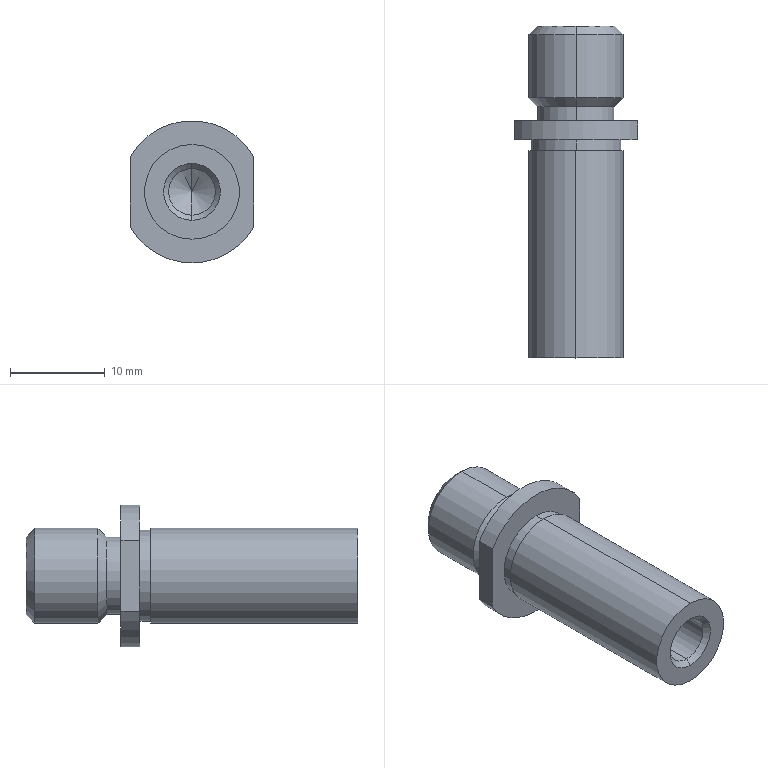Component | SolidWorks | MDJ12-10-Y2-F23-E10-N6.stp-1 | 1 solid | 28 faces | box 13 x 35 x 15 mm | volume 2570 mm3 | cylinder 13 | cone 8 | plane 7 | commonest cylinder face diameters 10 x4 15 x3 4.917 x2 8.16 x2 9.6 x2 | material 45
STEP:
#1=COLOUR_RGB('',0.7922,0.8196,0.9333);
#2=FILL_AREA_STYLE_COLOUR('',#1);
#3=FILL_AREA_STYLE('',(#2));
#4=SURFACE_STYLE_FILL_AREA(#3);
#5=SURFACE_SIDE_STYLE('',(#4));
#6=SURFACE_STYLE_USAGE(.BOTH.,#5);
#7=PRESENTATION_STYLE_ASSIGNMENT((#6));
#8=CARTESIAN_POINT('',(0.2836,0.06236,15.932));
#9=VERTEX_POINT('',#8);
#10=CARTESIAN_POINT('',(0.2836,0.06236,16.253));
#11=VERTEX_POINT('',#10);
#12=CARTESIAN_POINT('',(0.2836,0.06236,16.092));
#13=DIRECTION('',(-0.,-1.,0.));
#14=DIRECTION('',(-0.,0.,-1.));
#15=AXIS2_PLACEMENT_3D('',#12,#13,#14);
#16=CIRCLE('',#15,0.1606);
#17=EDGE_CURVE('',#9,#11,#16,.T.);
#18=ORIENTED_EDGE('',*,*,#17,.F.);
#19=CARTESIAN_POINT('',(0.2836,0.09858,15.896));
#20=VERTEX_POINT('',#19);
#21=CARTESIAN_POINT('',(0.2836,0.09858,15.896));
#22=DIRECTION('',(0.,0.7071,-0.7071));
#23=VECTOR('',#22,39.37);
#24=LINE('',#21,#23);
#25=EDGE_CURVE('',#9,#20,#24,.T.);
#26=ORIENTED_EDGE('',*,*,#25,.T.);
#27=CARTESIAN_POINT('',(0.2836,0.09858,16.289));
#28=VERTEX_POINT('',#27);
#29=CARTESIAN_POINT('',(0.2836,0.09858,16.092));
#30=DIRECTION('',(-0.,-1.,0.));
#31=DIRECTION('',(-0.,0.,-1.));
#32=AXIS2_PLACEMENT_3D('',#29,#30,#31);
#33=CIRCLE('',#32,0.1969);
#34=EDGE_CURVE('',#20,#28,#33,.T.);
#35=ORIENTED_EDGE('',*,*,#34,.T.);
#36=CARTESIAN_POINT('',(0.2836,0.09858,16.289));
#37=DIRECTION('',(0.,0.7071,0.7071));
#38=VECTOR('',#37,39.37);
#39=LINE('',#36,#38);
#40=EDGE_CURVE('',#11,#28,#39,.T.);
#41=ORIENTED_EDGE('',*,*,#40,.F.);
#42=EDGE_LOOP('',(#18,#26,#35,#41));
#43=FACE_OUTER_BOUND('',#42,.T.);
#44=CARTESIAN_POINT('',(0.2836,0.09858,16.092));
#45=DIRECTION('',(0.,1.,-0.));
#46=DIRECTION('',(0.,0.,1.));
#47=AXIS2_PLACEMENT_3D('',#44,#45,#46);
#48=CONICAL_SURFACE('',#47,0.1969,0.7854);
#49=ADVANCED_FACE('',(#43),#48,.T.);
#50=CARTESIAN_POINT('',(0.2836,-0.981,16.289));
#51=VERTEX_POINT('',#50);
#52=CARTESIAN_POINT('',(0.2836,-0.981,15.896));
#53=VERTEX_POINT('',#52);
#54=CARTESIAN_POINT('',(0.2836,-0.981,16.092));
#55=DIRECTION('',(-0.,-1.,0.));
#56=DIRECTION('',(-0.,0.,-1.));
#57=AXIS2_PLACEMENT_3D('',#54,#55,#56);
#58=CIRCLE('',#57,0.1969);
#59=EDGE_CURVE('',#51,#53,#58,.T.);
#60=ORIENTED_EDGE('',*,*,#59,.F.);
#61=CARTESIAN_POINT('',(0.2836,-0.1207,16.289));
#62=VERTEX_POINT('',#61);
#63=CARTESIAN_POINT('',(0.2836,-0.981,16.289));
#64=DIRECTION('',(0.,1.,-0.));
#65=VECTOR('',#64,39.37);
#66=LINE('',#63,#65);
#67=EDGE_CURVE('',#51,#62,#66,.T.);
#68=ORIENTED_EDGE('',*,*,#67,.T.);
#69=CARTESIAN_POINT('',(0.2836,-0.1207,15.896));
#70=VERTEX_POINT('',#69);
#71=CARTESIAN_POINT('',(0.2836,-0.1207,16.092));
#72=DIRECTION('',(-0.,-1.,0.));
#73=DIRECTION('',(-0.,0.,-1.));
#74=AXIS2_PLACEMENT_3D('',#71,#72,#73);
#75=CIRCLE('',#74,0.1969);
#76=EDGE_CURVE('',#62,#70,#75,.T.);
#77=ORIENTED_EDGE('',*,*,#76,.T.);
#78=CARTESIAN_POINT('',(0.2836,-0.981,15.896));
#79=DIRECTION('',(0.,1.,-0.));
#80=VECTOR('',#79,39.37);
#81=LINE('',#78,#80);
#82=EDGE_CURVE('',#53,#70,#81,.T.);
#83=ORIENTED_EDGE('',*,*,#82,.F.);
#84=EDGE_LOOP('',(#60,#68,#77,#83));
#85=FACE_OUTER_BOUND('',#84,.T.);
#86=CARTESIAN_POINT('',(0.2836,-0.981,16.092));
#87=DIRECTION('',(0.,1.,-0.));
#88=DIRECTION('',(-0.,0.,-1.));
#89=AXIS2_PLACEMENT_3D('',#86,#87,#88);
#90=CYLINDRICAL_SURFACE('',#89,0.1969);
#91=ADVANCED_FACE('',(#85),#90,.T.);
#92=CARTESIAN_POINT('',(0.2836,-0.9596,16.189));
#93=VERTEX_POINT('',#92);
#94=CARTESIAN_POINT('',(0.2836,-0.9596,15.996));
#95=VERTEX_POINT('',#94);
#96=CARTESIAN_POINT('',(0.2836,-0.9596,16.092));
#97=DIRECTION('',(-0.,-1.,0.));
#98=DIRECTION('',(-0.,0.,-1.));
#99=AXIS2_PLACEMENT_3D('',#96,#97,#98);
#100=CIRCLE('',#99,0.09679);
#101=EDGE_CURVE('',#93,#95,#100,.T.);
#102=ORIENTED_EDGE('',*,*,#101,.F.);
#103=CARTESIAN_POINT('',(0.2836,-0.981,16.211));
#104=VERTEX_POINT('',#103);
#105=CARTESIAN_POINT('',(0.2836,-0.981,16.211));
#106=DIRECTION('',(0.,-0.7071,0.7071));
#107=VECTOR('',#106,39.37);
#108=LINE('',#105,#107);
#109=EDGE_CURVE('',#93,#104,#108,.T.);
#110=ORIENTED_EDGE('',*,*,#109,.T.);
#111=CARTESIAN_POINT('',(0.2836,-0.981,15.974));
#112=VERTEX_POINT('',#111);
#113=CARTESIAN_POINT('',(0.2836,-0.981,16.092));
#114=DIRECTION('',(-0.,-1.,0.));
#115=DIRECTION('',(-0.,0.,-1.));
#116=AXIS2_PLACEMENT_3D('',#113,#114,#115);
#117=CIRCLE('',#116,0.1181);
#118=EDGE_CURVE('',#104,#112,#117,.T.);
#119=ORIENTED_EDGE('',*,*,#118,.T.);
#120=CARTESIAN_POINT('',(0.2836,-0.981,15.974));
#121=DIRECTION('',(-0.,-0.7071,-0.7071));
#122=VECTOR('',#121,39.37);
#123=LINE('',#120,#122);
#124=EDGE_CURVE('',#95,#112,#123,.T.);
#125=ORIENTED_EDGE('',*,*,#124,.F.);
#126=EDGE_LOOP('',(#102,#110,#119,#125));
#127=FACE_OUTER_BOUND('',#126,.T.);
#128=CARTESIAN_POINT('',(0.2836,-0.981,16.092));
#129=DIRECTION('',(-0.,-1.,0.));
#130=DIRECTION('',(-0.,0.,-1.));
#131=AXIS2_PLACEMENT_3D('',#128,#129,#130);
#132=CONICAL_SURFACE('',#131,0.1181,0.7854);
#133=ADVANCED_FACE('',(#127),#132,.F.);
#134=CARTESIAN_POINT('',(0.2836,-0.9596,16.092));
#135=DIRECTION('',(-0.,-1.,0.));
#136=DIRECTION('',(-0.,0.,-1.));
#137=AXIS2_PLACEMENT_3D('',#134,#135,#136);
#138=CIRCLE('',#137,0.09679);
#139=EDGE_CURVE('',#95,#93,#138,.T.);
#140=ORIENTED_EDGE('',*,*,#139,.T.);
#141=CARTESIAN_POINT('',(0.2836,-0.4175,16.189));
#142=VERTEX_POINT('',#141);
#143=CARTESIAN_POINT('',(0.2836,-0.981,16.189));
#144=DIRECTION('',(0.,1.,-0.));
#145=VECTOR('',#144,39.37);
#146=LINE('',#143,#145);
#147=EDGE_CURVE('',#93,#142,#146,.T.);
#148=ORIENTED_EDGE('',*,*,#147,.T.);
#149=CARTESIAN_POINT('',(0.2836,-0.4175,15.996));
#150=VERTEX_POINT('',#149);
#151=CARTESIAN_POINT('',(0.2836,-0.4175,16.092));
#152=DIRECTION('',(-0.,-1.,0.));
#153=DIRECTION('',(-0.,0.,-1.));
#154=AXIS2_PLACEMENT_3D('',#151,#152,#153);
#155=CIRCLE('',#154,0.09679);
#156=EDGE_CURVE('',#150,#142,#155,.T.);
#157=ORIENTED_EDGE('',*,*,#156,.F.);
#158=CARTESIAN_POINT('',(0.2836,-0.981,15.996));
#159=DIRECTION('',(0.,1.,-0.));
#160=VECTOR('',#159,39.37);
#161=LINE('',#158,#160);
#162=EDGE_CURVE('',#95,#150,#161,.T.);
#163=ORIENTED_EDGE('',*,*,#162,.F.);
#164=EDGE_LOOP('',(#140,#148,#157,#163));
#165=FACE_OUTER_BOUND('',#164,.T.);
#166=CARTESIAN_POINT('',(0.2836,-0.981,16.092));
#167=DIRECTION('',(0.,1.,-0.));
#168=DIRECTION('',(-0.,0.,-1.));
#169=AXIS2_PLACEMENT_3D('',#166,#167,#168);
#170=CYLINDRICAL_SURFACE('',#169,0.09679);
#171=ADVANCED_FACE('',(#165),#170,.F.);
#172=CARTESIAN_POINT('',(0.2836,-0.3616,16.092));
#173=VERTEX_POINT('',#172);
#174=CARTESIAN_POINT('',(0.2836,-0.4175,15.996));
#175=DIRECTION('',(-0.,-0.5,-0.866));
#176=VECTOR('',#175,39.37);
#177=LINE('',#174,#176);
#178=EDGE_CURVE('',#173,#150,#177,.T.);
#179=ORIENTED_EDGE('',*,*,#178,.F.);
#180=CARTESIAN_POINT('',(0.2836,-0.4175,16.189));
#181=DIRECTION('',(0.,-0.5,0.866));
#182=VECTOR('',#181,39.37);
#183=LINE('',#180,#182);
#184=EDGE_CURVE('',#173,#142,#183,.T.);
#185=ORIENTED_EDGE('',*,*,#184,.T.);
#186=CARTESIAN_POINT('',(0.2836,-0.4175,16.092));
#187=DIRECTION('',(-0.,-1.,0.));
#188=DIRECTION('',(-0.,0.,-1.));
#189=AXIS2_PLACEMENT_3D('',#186,#187,#188);
#190=CIRCLE('',#189,0.09679);
#191=EDGE_CURVE('',#142,#150,#190,.T.);
#192=ORIENTED_EDGE('',*,*,#191,.T.);
#193=EDGE_LOOP('',(#179,#185,#192));
#194=FACE_OUTER_BOUND('',#193,.T.);
#195=CARTESIAN_POINT('',(0.2836,-0.4175,16.092));
#196=DIRECTION('',(-0.,-1.,0.));
#197=DIRECTION('',(-0.,0.,-1.));
#198=AXIS2_PLACEMENT_3D('',#195,#196,#197);
#199=CONICAL_SURFACE('',#198,0.09679,1.047);
#200=ADVANCED_FACE('',(#194),#199,.F.);
#201=CARTESIAN_POINT('',(0.2836,0.003301,16.253));
#202=VERTEX_POINT('',#201);
#203=CARTESIAN_POINT('',(0.2836,0.003301,15.932));
#204=VERTEX_POINT('',#203);
#205=CARTESIAN_POINT('',(0.2836,0.003301,16.092));
#206=DIRECTION('',(-0.,-1.,0.));
#207=DIRECTION('',(-0.,0.,-1.));
#208=AXIS2_PLACEMENT_3D('',#205,#206,#207);
#209=CIRCLE('',#208,0.1606);
#210=EDGE_CURVE('',#202,#204,#209,.T.);
#211=ORIENTED_EDGE('',*,*,#210,.F.);
#212=CARTESIAN_POINT('',(0.2836,-0.981,16.253));
#213=DIRECTION('',(0.,1.,-0.));
#214=VECTOR('',#213,39.37);
#215=LINE('',#212,#214);
#216=EDGE_CURVE('',#202,#11,#215,.T.);
#217=ORIENTED_EDGE('',*,*,#216,.T.);
#218=CARTESIAN_POINT('',(0.2836,0.06236,16.092));
#219=DIRECTION('',(-0.,-1.,0.));
#220=DIRECTION('',(-0.,0.,-1.));
#221=AXIS2_PLACEMENT_3D('',#218,#219,#220);
#222=CIRCLE('',#221,0.1606);
#223=EDGE_CURVE('',#11,#9,#222,.T.);
#224=ORIENTED_EDGE('',*,*,#223,.T.);
#225=CARTESIAN_POINT('',(0.2836,-0.981,15.932));
#226=DIRECTION('',(0.,1.,-0.));
#227=VECTOR('',#226,39.37);
#228=LINE('',#225,#227);
#229=EDGE_CURVE('',#204,#9,#228,.T.);
#230=ORIENTED_EDGE('',*,*,#229,.F.);
#231=EDGE_LOOP('',(#211,#217,#224,#230));
#232=FACE_OUTER_BOUND('',#231,.T.);
#233=CARTESIAN_POINT('',(0.2836,-0.981,16.092));
#234=DIRECTION('',(0.,1.,-0.));
#235=DIRECTION('',(-0.,0.,-1.));
#236=AXIS2_PLACEMENT_3D('',#233,#234,#235);
#237=CYLINDRICAL_SURFACE('',#236,0.1606);
#238=ADVANCED_FACE('',(#232),#237,.T.);
#239=CARTESIAN_POINT('',(0.2836,-0.1207,16.281));
#240=VERTEX_POINT('',#239);
#241=CARTESIAN_POINT('',(0.2836,-0.1207,15.903));
#242=VERTEX_POINT('',#241);
#243=CARTESIAN_POINT('',(0.2836,-0.1207,16.092));
#244=DIRECTION('',(-0.,-1.,0.));
#245=DIRECTION('',(-0.,0.,-1.));
#246=AXIS2_PLACEMENT_3D('',#243,#244,#245);
#247=CIRCLE('',#246,0.189);
#248=EDGE_CURVE('',#240,#242,#247,.T.);
#249=ORIENTED_EDGE('',*,*,#248,.F.);
#250=CARTESIAN_POINT('',(0.2836,-0.07544,16.281));
#251=VERTEX_POINT('',#250);
#252=CARTESIAN_POINT('',(0.2836,-0.981,16.281));
#253=DIRECTION('',(0.,1.,-0.));
#254=VECTOR('',#253,39.37);
#255=LINE('',#252,#254);
#256=EDGE_CURVE('',#240,#251,#255,.T.);
#257=ORIENTED_EDGE('',*,*,#256,.T.);
#258=CARTESIAN_POINT('',(0.2836,-0.07544,15.903));
#259=VERTEX_POINT('',#258);
#260=CARTESIAN_POINT('',(0.2836,-0.07544,16.092));
#261=DIRECTION('',(-0.,-1.,0.));
#262=DIRECTION('',(-0.,0.,-1.));
#263=AXIS2_PLACEMENT_3D('',#260,#261,#262);
#264=CIRCLE('',#263,0.189);
#265=EDGE_CURVE('',#251,#259,#264,.T.);
#266=ORIENTED_EDGE('',*,*,#265,.T.);
#267=CARTESIAN_POINT('',(0.2836,-0.981,15.903));
#268=DIRECTION('',(0.,1.,-0.));
#269=VECTOR('',#268,39.37);
#270=LINE('',#267,#269);
#271=EDGE_CURVE('',#242,#259,#270,.T.);
#272=ORIENTED_EDGE('',*,*,#271,.F.);
#273=EDGE_LOOP('',(#249,#257,#266,#272));
#274=FACE_OUTER_BOUND('',#273,.T.);
#275=CARTESIAN_POINT('',(0.2836,-0.981,16.092));
#276=DIRECTION('',(0.,1.,-0.));
#277=DIRECTION('',(-0.,0.,-1.));
#278=AXIS2_PLACEMENT_3D('',#275,#276,#277);
#279=CYLINDRICAL_SURFACE('',#278,0.189);
#280=ADVANCED_FACE('',(#274),#279,.T.);
#281=CARTESIAN_POINT('',(0.2836,-0.07544,15.797));
#282=VERTEX_POINT('',#281);
#283=CARTESIAN_POINT('',(0.5395,-0.07544,15.945));
#284=VERTEX_POINT('',#283);
#285=CARTESIAN_POINT('',(0.2836,-0.07544,16.092));
#286=DIRECTION('',(-0.,-1.,0.));
#287=DIRECTION('',(-0.,0.,-1.));
#288=AXIS2_PLACEMENT_3D('',#285,#286,#287);
#289=CIRCLE('',#288,0.2953);
#290=EDGE_CURVE('',#282,#284,#289,.T.);
#291=ORIENTED_EDGE('',*,*,#290,.F.);
#292=CARTESIAN_POINT('',(0.2836,0.003301,15.797));
#293=VERTEX_POINT('',#292);
#294=CARTESIAN_POINT('',(0.2836,-0.981,15.797));
#295=DIRECTION('',(0.,1.,-0.));
#296=VECTOR('',#295,39.37);
#297=LINE('',#294,#296);
#298=EDGE_CURVE('',#282,#293,#297,.T.);
#299=ORIENTED_EDGE('',*,*,#298,.T.);
#300=CARTESIAN_POINT('',(0.5395,0.003301,15.945));
#301=VERTEX_POINT('',#300);
#302=CARTESIAN_POINT('',(0.2836,0.003301,16.092));
#303=DIRECTION('',(-0.,-1.,0.));
#304=DIRECTION('',(-0.,0.,-1.));
#305=AXIS2_PLACEMENT_3D('',#302,#303,#304);
#306=CIRCLE('',#305,0.2953);
#307=EDGE_CURVE('',#293,#301,#306,.T.);
#308=ORIENTED_EDGE('',*,*,#307,.T.);
#309=CARTESIAN_POINT('',(0.5395,-0.981,15.945));
#310=DIRECTION('',(-0.,-1.,0.));
#311=VECTOR('',#310,39.37);
#312=LINE('',#309,#311);
#313=EDGE_CURVE('',#301,#284,#312,.T.);
#314=ORIENTED_EDGE('',*,*,#313,.T.);
#315=EDGE_LOOP('',(#291,#299,#308,#314));
#316=FACE_OUTER_BOUND('',#315,.T.);
#317=CARTESIAN_POINT('',(0.2836,-0.981,16.092));
#318=DIRECTION('',(0.,1.,-0.));
#319=DIRECTION('',(-0.,0.,-1.));
#320=AXIS2_PLACEMENT_3D('',#317,#318,#319);
#321=CYLINDRICAL_SURFACE('',#320,0.2953);
#322=ADVANCED_FACE('',(#316),#321,.T.);
#323=CARTESIAN_POINT('',(0.2836,0.397,15.932));
#324=VERTEX_POINT('',#323);
#325=CARTESIAN_POINT('',(0.2836,0.397,16.253));
#326=VERTEX_POINT('',#325);
#327=CARTESIAN_POINT('',(0.2836,0.397,16.092));
#328=DIRECTION('',(-0.,-1.,0.));
#329=DIRECTION('',(-0.,0.,-1.));
#330=AXIS2_PLACEMENT_3D('',#327,#328,#329);
#331=CIRCLE('',#330,0.1606);
#332=EDGE_CURVE('',#324,#326,#331,.T.);
#333=ORIENTED_EDGE('',*,*,#332,.T.);
#334=CARTESIAN_POINT('',(0.2836,0.3608,16.289));
#335=VERTEX_POINT('',#334);
#336=CARTESIAN_POINT('',(0.2836,0.397,16.253));
#337=DIRECTION('',(0.,-0.7071,0.7071));
#338=VECTOR('',#337,39.37);
#339=LINE('',#336,#338);
#340=EDGE_CURVE('',#326,#335,#339,.T.);
#341=ORIENTED_EDGE('',*,*,#340,.T.);
#342=CARTESIAN_POINT('',(0.2836,0.3608,15.896));
#343=VERTEX_POINT('',#342);
#344=CARTESIAN_POINT('',(0.2836,0.3608,16.092));
#345=DIRECTION('',(-0.,-1.,0.));
#346=DIRECTION('',(-0.,0.,-1.));
#347=AXIS2_PLACEMENT_3D('',#344,#345,#346);
#348=CIRCLE('',#347,0.1969);
#349=EDGE_CURVE('',#343,#335,#348,.T.);
#350=ORIENTED_EDGE('',*,*,#349,.F.);
#351=CARTESIAN_POINT('',(0.2836,0.397,15.932));
#352=DIRECTION('',(-0.,-0.7071,-0.7071));
#353=VECTOR('',#352,39.37);
#354=LINE('',#351,#353);
#355=EDGE_CURVE('',#324,#343,#354,.T.);
#356=ORIENTED_EDGE('',*,*,#355,.F.);
#357=EDGE_LOOP('',(#333,#341,#350,#356));
#358=FACE_OUTER_BOUND('',#357,.T.);
#359=CARTESIAN_POINT('',(0.2836,0.397,16.092));
#360=DIRECTION('',(-0.,-1.,0.));
#361=DIRECTION('',(-0.,0.,-1.));
#362=AXIS2_PLACEMENT_3D('',#359,#360,#361);
#363=CONICAL_SURFACE('',#362,0.1606,0.7854);
#364=ADVANCED_FACE('',(#358),#363,.T.);
#365=CARTESIAN_POINT('',(0.2836,0.09858,16.092));
#366=DIRECTION('',(-0.,-1.,0.));
#367=DIRECTION('',(-0.,0.,-1.));
#368=AXIS2_PLACEMENT_3D('',#365,#366,#367);
#369=CIRCLE('',#368,0.1969);
#370=EDGE_CURVE('',#28,#20,#369,.T.);
#371=ORIENTED_EDGE('',*,*,#370,.F.);
#372=CARTESIAN_POINT('',(0.2836,-0.981,16.289));
#373=DIRECTION('',(0.,1.,-0.));
#374=VECTOR('',#373,39.37);
#375=LINE('',#372,#374);
#376=EDGE_CURVE('',#28,#335,#375,.T.);
#377=ORIENTED_EDGE('',*,*,#376,.T.);
#378=CARTESIAN_POINT('',(0.2836,0.3608,16.092));
#379=DIRECTION('',(-0.,-1.,0.));
#380=DIRECTION('',(-0.,0.,-1.));
#381=AXIS2_PLACEMENT_3D('',#378,#379,#380);
#382=CIRCLE('',#381,0.1969);
#383=EDGE_CURVE('',#335,#343,#382,.T.);
#384=ORIENTED_EDGE('',*,*,#383,.T.);
#385=CARTESIAN_POINT('',(0.2836,-0.981,15.896));
#386=DIRECTION('',(0.,1.,-0.));
#387=VECTOR('',#386,39.37);
#388=LINE('',#385,#387);
#389=EDGE_CURVE('',#20,#343,#388,.T.);
#390=ORIENTED_EDGE('',*,*,#389,.F.);
#391=EDGE_LOOP('',(#371,#377,#384,#390));
#392=FACE_OUTER_BOUND('',#391,.T.);
#393=CARTESIAN_POINT('',(0.2836,-0.981,16.092));
#394=DIRECTION('',(0.,1.,-0.));
#395=DIRECTION('',(-0.,0.,-1.));
#396=AXIS2_PLACEMENT_3D('',#393,#394,#395);
#397=CYLINDRICAL_SURFACE('',#396,0.1969);
#398=ADVANCED_FACE('',(#392),#397,.T.);
#399=CARTESIAN_POINT('',(0.5395,0.003301,16.24));
#400=VERTEX_POINT('',#399);
#401=CARTESIAN_POINT('',(0.02769,0.003301,16.24));
#402=VERTEX_POINT('',#401);
#403=CARTESIAN_POINT('',(0.2836,0.003301,16.092));
#404=DIRECTION('',(-0.,-1.,0.));
#405=DIRECTION('',(-0.,0.,-1.));
#406=AXIS2_PLACEMENT_3D('',#403,#404,#405);
#407=CIRCLE('',#406,0.2953);
#408=EDGE_CURVE('',#400,#402,#407,.T.);
#409=ORIENTED_EDGE('',*,*,#408,.T.);
#410=CARTESIAN_POINT('',(0.02769,-0.07544,16.24));
#411=VERTEX_POINT('',#410);
#412=CARTESIAN_POINT('',(0.02769,-0.981,16.24));
#413=DIRECTION('',(-0.,-1.,0.));
#414=VECTOR('',#413,39.37);
#415=LINE('',#412,#414);
#416=EDGE_CURVE('',#402,#411,#415,.T.);
#417=ORIENTED_EDGE('',*,*,#416,.T.);
#418=CARTESIAN_POINT('',(0.5395,-0.07544,16.24));
#419=VERTEX_POINT('',#418);
#420=CARTESIAN_POINT('',(0.2836,-0.07544,16.092));
#421=DIRECTION('',(-0.,-1.,0.));
#422=DIRECTION('',(-0.,0.,-1.));
#423=AXIS2_PLACEMENT_3D('',#420,#421,#422);
#424=CIRCLE('',#423,0.2953);
#425=EDGE_CURVE('',#419,#411,#424,.T.);
#426=ORIENTED_EDGE('',*,*,#425,.F.);
#427=CARTESIAN_POINT('',(0.5395,-0.981,16.24));
#428=DIRECTION('',(0.,1.,-0.));
#429=VECTOR('',#428,39.37);
#430=LINE('',#427,#429);
#431=EDGE_CURVE('',#419,#400,#430,.T.);
#432=ORIENTED_EDGE('',*,*,#431,.T.);
#433=EDGE_LOOP('',(#409,#417,#426,#432));
#434=FACE_OUTER_BOUND('',#433,.T.);
#435=CARTESIAN_POINT('',(0.2836,-0.981,16.092));
#436=DIRECTION('',(0.,1.,-0.));
#437=DIRECTION('',(-0.,0.,-1.));
#438=AXIS2_PLACEMENT_3D('',#435,#436,#437);
#439=CYLINDRICAL_SURFACE('',#438,0.2953);
#440=ADVANCED_FACE('',(#434),#439,.T.);
#441=ORIENTED_EDGE('',*,*,#332,.F.);
#442=CARTESIAN_POINT('',(0.2836,0.397,16.092));
#443=DIRECTION('',(-0.,-1.,0.));
#444=DIRECTION('',(-0.,0.,-1.));
#445=AXIS2_PLACEMENT_3D('',#442,#443,#444);
#446=CIRCLE('',#445,0.1606);
#447=EDGE_CURVE('',#326,#324,#446,.T.);
#448=ORIENTED_EDGE('',*,*,#447,.F.);
#449=EDGE_LOOP('',(#441,#448));
#450=FACE_OUTER_BOUND('',#449,.T.);
#451=CARTESIAN_POINT('',(0.2836,0.397,16.092));
#452=DIRECTION('',(-0.,-1.,0.));
#453=DIRECTION('',(-1.,0.,0.));
#454=AXIS2_PLACEMENT_3D('',#451,#452,#453);
#455=PLANE('',#454);
#456=ADVANCED_FACE('',(#450),#455,.F.);
#457=CARTESIAN_POINT('',(0.02769,0.003301,15.945));
#458=VERTEX_POINT('',#457);
#459=CARTESIAN_POINT('',(0.02769,0.003301,16.388));
#460=DIRECTION('',(-0.,-0.,-1.));
#461=VECTOR('',#460,39.37);
#462=LINE('',#459,#461);
#463=EDGE_CURVE('',#402,#458,#462,.T.);
#464=ORIENTED_EDGE('',*,*,#463,.T.);
#465=CARTESIAN_POINT('',(0.02769,-0.07544,15.945));
#466=VERTEX_POINT('',#465);
#467=CARTESIAN_POINT('',(0.02769,-0.981,15.945));
#468=DIRECTION('',(0.,1.,-0.));
#469=VECTOR('',#468,39.37);
#470=LINE('',#467,#469);
#471=EDGE_CURVE('',#466,#458,#470,.T.);
#472=ORIENTED_EDGE('',*,*,#471,.F.);
#473=CARTESIAN_POINT('',(0.02769,-0.07544,16.388));
#474=DIRECTION('',(-0.,-0.,-1.));
#475=VECTOR('',#474,39.37);
#476=LINE('',#473,#475);
#477=EDGE_CURVE('',#411,#466,#476,.T.);
#478=ORIENTED_EDGE('',*,*,#477,.F.);
#479=ORIENTED_EDGE('',*,*,#416,.F.);
#480=EDGE_LOOP('',(#464,#472,#478,#479));
#481=FACE_OUTER_BOUND('',#480,.T.);
#482=CARTESIAN_POINT('',(0.02769,-0.07544,16.388));
#483=DIRECTION('',(1.,-0.,-0.));
#484=DIRECTION('',(-0.,-0.,-1.));
#485=AXIS2_PLACEMENT_3D('',#482,#483,#484);
#486=PLANE('',#485);
#487=ADVANCED_FACE('',(#481),#486,.F.);
#488=CARTESIAN_POINT('',(0.2836,0.003301,16.092));
#489=DIRECTION('',(-0.,-1.,0.));
#490=DIRECTION('',(-0.,0.,-1.));
#491=AXIS2_PLACEMENT_3D('',#488,#489,#490);
#492=CIRCLE('',#491,0.2953);
#493=EDGE_CURVE('',#458,#293,#492,.T.);
#494=ORIENTED_EDGE('',*,*,#493,.F.);
#495=ORIENTED_EDGE('',*,*,#463,.F.);
#496=ORIENTED_EDGE('',*,*,#408,.F.);
#497=CARTESIAN_POINT('',(0.5395,0.003301,15.797));
#498=DIRECTION('',(0.,0.,1.));
#499=VECTOR('',#498,39.37);
#500=LINE('',#497,#499);
#501=EDGE_CURVE('',#301,#400,#500,.T.);
#502=ORIENTED_EDGE('',*,*,#501,.F.);
#503=ORIENTED_EDGE('',*,*,#307,.F.);
#504=EDGE_LOOP('',(#494,#495,#496,#502,#503));
#505=FACE_OUTER_BOUND('',#504,.T.);
#506=CARTESIAN_POINT('',(0.2836,0.003301,16.092));
#507=DIRECTION('',(-0.,-1.,0.));
#508=DIRECTION('',(-0.,0.,-1.));
#509=AXIS2_PLACEMENT_3D('',#506,#507,#508);
#510=CIRCLE('',#509,0.1606);
#511=EDGE_CURVE('',#204,#202,#510,.T.);
#512=ORIENTED_EDGE('',*,*,#511,.T.);
#513=ORIENTED_EDGE('',*,*,#210,.T.);
#514=EDGE_LOOP('',(#512,#513));
#515=FACE_BOUND('',#514,.T.);
#516=CARTESIAN_POINT('',(0.2836,0.003301,15.932));
#517=DIRECTION('',(-0.,-1.,0.));
#518=DIRECTION('',(-1.,0.,0.));
#519=AXIS2_PLACEMENT_3D('',#516,#517,#518);
#520=PLANE('',#519);
#521=ADVANCED_FACE('',(#505,#515),#520,.F.);
#522=ORIENTED_EDGE('',*,*,#376,.F.);
#523=ORIENTED_EDGE('',*,*,#34,.F.);
#524=ORIENTED_EDGE('',*,*,#389,.T.);
#525=ORIENTED_EDGE('',*,*,#349,.T.);
#526=EDGE_LOOP('',(#522,#523,#524,#525));
#527=FACE_OUTER_BOUND('',#526,.T.);
#528=CARTESIAN_POINT('',(0.2836,-0.981,16.092));
#529=DIRECTION('',(0.,1.,-0.));
#530=DIRECTION('',(-0.,0.,-1.));
#531=AXIS2_PLACEMENT_3D('',#528,#529,#530);
#532=CYLINDRICAL_SURFACE('',#531,0.1969);
#533=ADVANCED_FACE('',(#527),#532,.T.);
#534=ORIENTED_EDGE('',*,*,#340,.F.);
#535=ORIENTED_EDGE('',*,*,#447,.T.);
#536=ORIENTED_EDGE('',*,*,#355,.T.);
#537=ORIENTED_EDGE('',*,*,#383,.F.);
#538=EDGE_LOOP('',(#534,#535,#536,#537));
#539=FACE_OUTER_BOUND('',#538,.T.);
#540=CARTESIAN_POINT('',(0.2836,0.397,16.092));
#541=DIRECTION('',(-0.,-1.,0.));
#542=DIRECTION('',(-0.,0.,-1.));
#543=AXIS2_PLACEMENT_3D('',#540,#541,#542);
#544=CONICAL_SURFACE('',#543,0.1606,0.7854);
#545=ADVANCED_FACE('',(#539),#544,.T.);
#546=ORIENTED_EDGE('',*,*,#298,.F.);
#547=CARTESIAN_POINT('',(0.2836,-0.07544,16.092));
#548=DIRECTION('',(-0.,-1.,0.));
#549=DIRECTION('',(-0.,0.,-1.));
#550=AXIS2_PLACEMENT_3D('',#547,#548,#549);
#551=CIRCLE('',#550,0.2953);
#552=EDGE_CURVE('',#466,#282,#551,.T.);
#553=ORIENTED_EDGE('',*,*,#552,.F.);
#554=ORIENTED_EDGE('',*,*,#471,.T.);
#555=ORIENTED_EDGE('',*,*,#493,.T.);
#556=EDGE_LOOP('',(#546,#553,#554,#555));
#557=FACE_OUTER_BOUND('',#556,.T.);
#558=CARTESIAN_POINT('',(0.2836,-0.981,16.092));
#559=DIRECTION('',(0.,1.,-0.));
#560=DIRECTION('',(-0.,0.,-1.));
#561=AXIS2_PLACEMENT_3D('',#558,#559,#560);
#562=CYLINDRICAL_SURFACE('',#561,0.2953);
#563=ADVANCED_FACE('',(#557),#562,.T.);
#564=ORIENTED_EDGE('',*,*,#425,.T.);
#565=ORIENTED_EDGE('',*,*,#477,.T.);
#566=ORIENTED_EDGE('',*,*,#552,.T.);
#567=ORIENTED_EDGE('',*,*,#290,.T.);
#568=CARTESIAN_POINT('',(0.5395,-0.07544,15.797));
#569=DIRECTION('',(0.,0.,1.));
#570=VECTOR('',#569,39.37);
#571=LINE('',#568,#570);
#572=EDGE_CURVE('',#284,#419,#571,.T.);
#573=ORIENTED_EDGE('',*,*,#572,.T.);
#574=EDGE_LOOP('',(#564,#565,#566,#567,#573));
#575=FACE_OUTER_BOUND('',#574,.T.);
#576=CARTESIAN_POINT('',(0.2836,-0.07544,16.092));
#577=DIRECTION('',(-0.,-1.,0.));
#578=DIRECTION('',(-0.,0.,-1.));
#579=AXIS2_PLACEMENT_3D('',#576,#577,#578);
#580=CIRCLE('',#579,0.189);
#581=EDGE_CURVE('',#259,#251,#580,.T.);
#582=ORIENTED_EDGE('',*,*,#581,.F.);
#583=ORIENTED_EDGE('',*,*,#265,.F.);
#584=EDGE_LOOP('',(#582,#583));
#585=FACE_BOUND('',#584,.T.);
#586=CARTESIAN_POINT('',(0.2836,-0.07544,15.797));
#587=DIRECTION('',(0.,1.,-0.));
#588=DIRECTION('',(1.,-0.,-0.));
#589=AXIS2_PLACEMENT_3D('',#586,#587,#588);
#590=PLANE('',#589);
#591=ADVANCED_FACE('',(#575,#585),#590,.F.);
#592=ORIENTED_EDGE('',*,*,#256,.F.);
#593=CARTESIAN_POINT('',(0.2836,-0.1207,16.092));
#594=DIRECTION('',(-0.,-1.,0.));
#595=DIRECTION('',(-0.,0.,-1.));
#596=AXIS2_PLACEMENT_3D('',#593,#594,#595);
#597=CIRCLE('',#596,0.189);
#598=EDGE_CURVE('',#242,#240,#597,.T.);
#599=ORIENTED_EDGE('',*,*,#598,.F.);
#600=ORIENTED_EDGE('',*,*,#271,.T.);
#601=ORIENTED_EDGE('',*,*,#581,.T.);
#602=EDGE_LOOP('',(#592,#599,#600,#601));
#603=FACE_OUTER_BOUND('',#602,.T.);
#604=CARTESIAN_POINT('',(0.2836,-0.981,16.092));
#605=DIRECTION('',(0.,1.,-0.));
#606=DIRECTION('',(-0.,0.,-1.));
#607=AXIS2_PLACEMENT_3D('',#604,#605,#606);
#608=CYLINDRICAL_SURFACE('',#607,0.189);
#609=ADVANCED_FACE('',(#603),#608,.T.);
#610=ORIENTED_EDGE('',*,*,#216,.F.);
#611=ORIENTED_EDGE('',*,*,#511,.F.);
#612=ORIENTED_EDGE('',*,*,#229,.T.);
#613=ORIENTED_EDGE('',*,*,#17,.T.);
#614=EDGE_LOOP('',(#610,#611,#612,#613));
#615=FACE_OUTER_BOUND('',#614,.T.);
#616=CARTESIAN_POINT('',(0.2836,-0.981,16.092));
#617=DIRECTION('',(0.,1.,-0.));
#618=DIRECTION('',(-0.,0.,-1.));
#619=AXIS2_PLACEMENT_3D('',#616,#617,#618);
#620=CYLINDRICAL_SURFACE('',#619,0.1606);
#621=ADVANCED_FACE('',(#615),#620,.T.);
#622=ORIENTED_EDGE('',*,*,#501,.T.);
#623=ORIENTED_EDGE('',*,*,#431,.F.);
#624=ORIENTED_EDGE('',*,*,#572,.F.);
#625=ORIENTED_EDGE('',*,*,#313,.F.);
#626=EDGE_LOOP('',(#622,#623,#624,#625));
#627=FACE_OUTER_BOUND('',#626,.T.);
#628=CARTESIAN_POINT('',(0.5395,-0.07544,15.797));
#629=DIRECTION('',(-1.,0.,0.));
#630=DIRECTION('',(0.,1.,-0.));
#631=AXIS2_PLACEMENT_3D('',#628,#629,#630);
#632=PLANE('',#631);
#633=ADVANCED_FACE('',(#627),#632,.F.);
#634=ORIENTED_EDGE('',*,*,#184,.F.);
#635=ORIENTED_EDGE('',*,*,#178,.T.);
#636=ORIENTED_EDGE('',*,*,#156,.T.);
#637=EDGE_LOOP('',(#634,#635,#636));
#638=FACE_OUTER_BOUND('',#637,.T.);
#639=CARTESIAN_POINT('',(0.2836,-0.4175,16.092));
#640=DIRECTION('',(-0.,-1.,0.));
#641=DIRECTION('',(-0.,0.,-1.));
#642=AXIS2_PLACEMENT_3D('',#639,#640,#641);
#643=CONICAL_SURFACE('',#642,0.09679,1.047);
#644=ADVANCED_FACE('',(#638),#643,.F.);
#645=ORIENTED_EDGE('',*,*,#147,.F.);
#646=ORIENTED_EDGE('',*,*,#101,.T.);
#647=ORIENTED_EDGE('',*,*,#162,.T.);
#648=ORIENTED_EDGE('',*,*,#191,.F.);
#649=EDGE_LOOP('',(#645,#646,#647,#648));
#650=FACE_OUTER_BOUND('',#649,.T.);
#651=CARTESIAN_POINT('',(0.2836,-0.981,16.092));
#652=DIRECTION('',(0.,1.,-0.));
#653=DIRECTION('',(-0.,0.,-1.));
#654=AXIS2_PLACEMENT_3D('',#651,#652,#653);
#655=CYLINDRICAL_SURFACE('',#654,0.09679);
#656=ADVANCED_FACE('',(#650),#655,.F.);
#657=ORIENTED_EDGE('',*,*,#109,.F.);
#658=ORIENTED_EDGE('',*,*,#139,.F.);
#659=ORIENTED_EDGE('',*,*,#124,.T.);
#660=CARTESIAN_POINT('',(0.2836,-0.981,16.092));
#661=DIRECTION('',(-0.,-1.,0.));
#662=DIRECTION('',(-0.,0.,-1.));
#663=AXIS2_PLACEMENT_3D('',#660,#661,#662);
#664=CIRCLE('',#663,0.1181);
#665=EDGE_CURVE('',#112,#104,#664,.T.);
#666=ORIENTED_EDGE('',*,*,#665,.T.);
#667=EDGE_LOOP('',(#657,#658,#659,#666));
#668=FACE_OUTER_BOUND('',#667,.T.);
#669=CARTESIAN_POINT('',(0.2836,-0.981,16.092));
#670=DIRECTION('',(-0.,-1.,0.));
#671=DIRECTION('',(-0.,0.,-1.));
#672=AXIS2_PLACEMENT_3D('',#669,#670,#671);
#673=CONICAL_SURFACE('',#672,0.1181,0.7854);
#674=ADVANCED_FACE('',(#668),#673,.F.);
#675=CARTESIAN_POINT('',(0.2836,-0.981,16.092));
#676=DIRECTION('',(-0.,-1.,0.));
#677=DIRECTION('',(-0.,0.,-1.));
#678=AXIS2_PLACEMENT_3D('',#675,#676,#677);
#679=CIRCLE('',#678,0.1969);
#680=EDGE_CURVE('',#53,#51,#679,.T.);
#681=ORIENTED_EDGE('',*,*,#680,.T.);
#682=ORIENTED_EDGE('',*,*,#59,.T.);
#683=EDGE_LOOP('',(#681,#682));
#684=FACE_OUTER_BOUND('',#683,.T.);
#685=ORIENTED_EDGE('',*,*,#665,.F.);
#686=ORIENTED_EDGE('',*,*,#118,.F.);
#687=EDGE_LOOP('',(#685,#686));
#688=FACE_BOUND('',#687,.T.);
#689=CARTESIAN_POINT('',(0.2836,-0.981,15.896));
#690=DIRECTION('',(0.,1.,-0.));
#691=DIRECTION('',(1.,-0.,-0.));
#692=AXIS2_PLACEMENT_3D('',#689,#690,#691);
#693=PLANE('',#692);
#694=ADVANCED_FACE('',(#684,#688),#693,.F.);
#695=ORIENTED_EDGE('',*,*,#67,.F.);
#696=ORIENTED_EDGE('',*,*,#680,.F.);
#697=ORIENTED_EDGE('',*,*,#82,.T.);
#698=CARTESIAN_POINT('',(0.2836,-0.1207,16.092));
#699=DIRECTION('',(-0.,-1.,0.));
#700=DIRECTION('',(-0.,0.,-1.));
#701=AXIS2_PLACEMENT_3D('',#698,#699,#700);
#702=CIRCLE('',#701,0.1969);
#703=EDGE_CURVE('',#70,#62,#702,.T.);
#704=ORIENTED_EDGE('',*,*,#703,.T.);
#705=EDGE_LOOP('',(#695,#696,#697,#704));
#706=FACE_OUTER_BOUND('',#705,.T.);
#707=CARTESIAN_POINT('',(0.2836,-0.981,16.092));
#708=DIRECTION('',(0.,1.,-0.));
#709=DIRECTION('',(-0.,0.,-1.));
#710=AXIS2_PLACEMENT_3D('',#707,#708,#709);
#711=CYLINDRICAL_SURFACE('',#710,0.1969);
#712=ADVANCED_FACE('',(#706),#711,.T.);
#713=ORIENTED_EDGE('',*,*,#703,.F.);
#714=ORIENTED_EDGE('',*,*,#76,.F.);
#715=EDGE_LOOP('',(#713,#714));
#716=FACE_OUTER_BOUND('',#715,.T.);
#717=ORIENTED_EDGE('',*,*,#598,.T.);
#718=ORIENTED_EDGE('',*,*,#248,.T.);
#719=EDGE_LOOP('',(#717,#718));
#720=FACE_BOUND('',#719,.T.);
#721=CARTESIAN_POINT('',(0.2836,-0.1207,15.903));
#722=DIRECTION('',(-0.,-1.,0.));
#723=DIRECTION('',(-1.,0.,0.));
#724=AXIS2_PLACEMENT_3D('',#721,#722,#723);
#725=PLANE('',#724);
#726=ADVANCED_FACE('',(#716,#720),#725,.F.);
#727=ORIENTED_EDGE('',*,*,#25,.F.);
#728=ORIENTED_EDGE('',*,*,#223,.F.);
#729=ORIENTED_EDGE('',*,*,#40,.T.);
#730=ORIENTED_EDGE('',*,*,#370,.T.);
#731=EDGE_LOOP('',(#727,#728,#729,#730));
#732=FACE_OUTER_BOUND('',#731,.T.);
#733=CARTESIAN_POINT('',(0.2836,0.09858,16.092));
#734=DIRECTION('',(0.,1.,-0.));
#735=DIRECTION('',(0.,0.,1.));
#736=AXIS2_PLACEMENT_3D('',#733,#734,#735);
#737=CONICAL_SURFACE('',#736,0.1969,0.7854);
#738=ADVANCED_FACE('',(#732),#737,.T.);
#739=CLOSED_SHELL('',(#49,#91,#133,#171,#200,#238,#280,#322,#364,#398,#440,#456,#487,#521,#533,#545,#563,#591,#609,#621,#633,#644,#656,#674,#694,#712,#726,#738));
#740=MANIFOLD_SOLID_BREP('',#739);
#741=STYLED_ITEM('',(#7),#740);
#742=PRESENTATION_LAYER_ASSIGNMENT('','',(#741));
#743=(LENGTH_UNIT()NAMED_UNIT(*)SI_UNIT($,.METRE.));
#744=LENGTH_MEASURE_WITH_UNIT(LENGTH_MEASURE(0.0254),#743);
#745=DIMENSIONAL_EXPONENTS(1.,0.,0.,0.,0.,0.,0.);
#746=(CONVERSION_BASED_UNIT('',#744)LENGTH_UNIT()NAMED_UNIT(#745));
#747=UNCERTAINTY_MEASURE_WITH_UNIT(LENGTH_MEASURE(0.00001),#746,'','');
#748=(NAMED_UNIT(*)PLANE_ANGLE_UNIT()SI_UNIT($,.RADIAN.));
#749=(NAMED_UNIT(*)SI_UNIT($,.STERADIAN.)SOLID_ANGLE_UNIT());
#750=(GEOMETRIC_REPRESENTATION_CONTEXT(3)GLOBAL_UNCERTAINTY_ASSIGNED_CONTEXT((#747))GLOBAL_UNIT_ASSIGNED_CONTEXT((#746,#748,#749))REPRESENTATION_CONTEXT('',''));
#751=MECHANICAL_DESIGN_GEOMETRIC_PRESENTATION_REPRESENTATION('',(#741),#750);
#752=CARTESIAN_POINT('',(0.,0.,0.));
#753=DIRECTION('',(0.,0.,1.));
#754=DIRECTION('',(1.,0.,0.));
#755=AXIS2_PLACEMENT_3D('',#752,#753,#754);
#756=(LENGTH_UNIT()NAMED_UNIT(*)SI_UNIT($,.METRE.));
#757=LENGTH_MEASURE_WITH_UNIT(LENGTH_MEASURE(0.0254),#756);
#758=DIMENSIONAL_EXPONENTS(1.,0.,0.,0.,0.,0.,0.);
#759=(CONVERSION_BASED_UNIT('',#757)LENGTH_UNIT()NAMED_UNIT(#758));
#760=UNCERTAINTY_MEASURE_WITH_UNIT(LENGTH_MEASURE(0.00001),#759,'','');
#761=(NAMED_UNIT(*)PLANE_ANGLE_UNIT()SI_UNIT($,.RADIAN.));
#762=(NAMED_UNIT(*)SI_UNIT($,.STERADIAN.)SOLID_ANGLE_UNIT());
#763=(GEOMETRIC_REPRESENTATION_CONTEXT(3)GLOBAL_UNCERTAINTY_ASSIGNED_CONTEXT((#760))GLOBAL_UNIT_ASSIGNED_CONTEXT((#759,#761,#762))REPRESENTATION_CONTEXT('',''));
#764=ADVANCED_BREP_SHAPE_REPRESENTATION('',(#740,#755),#763);